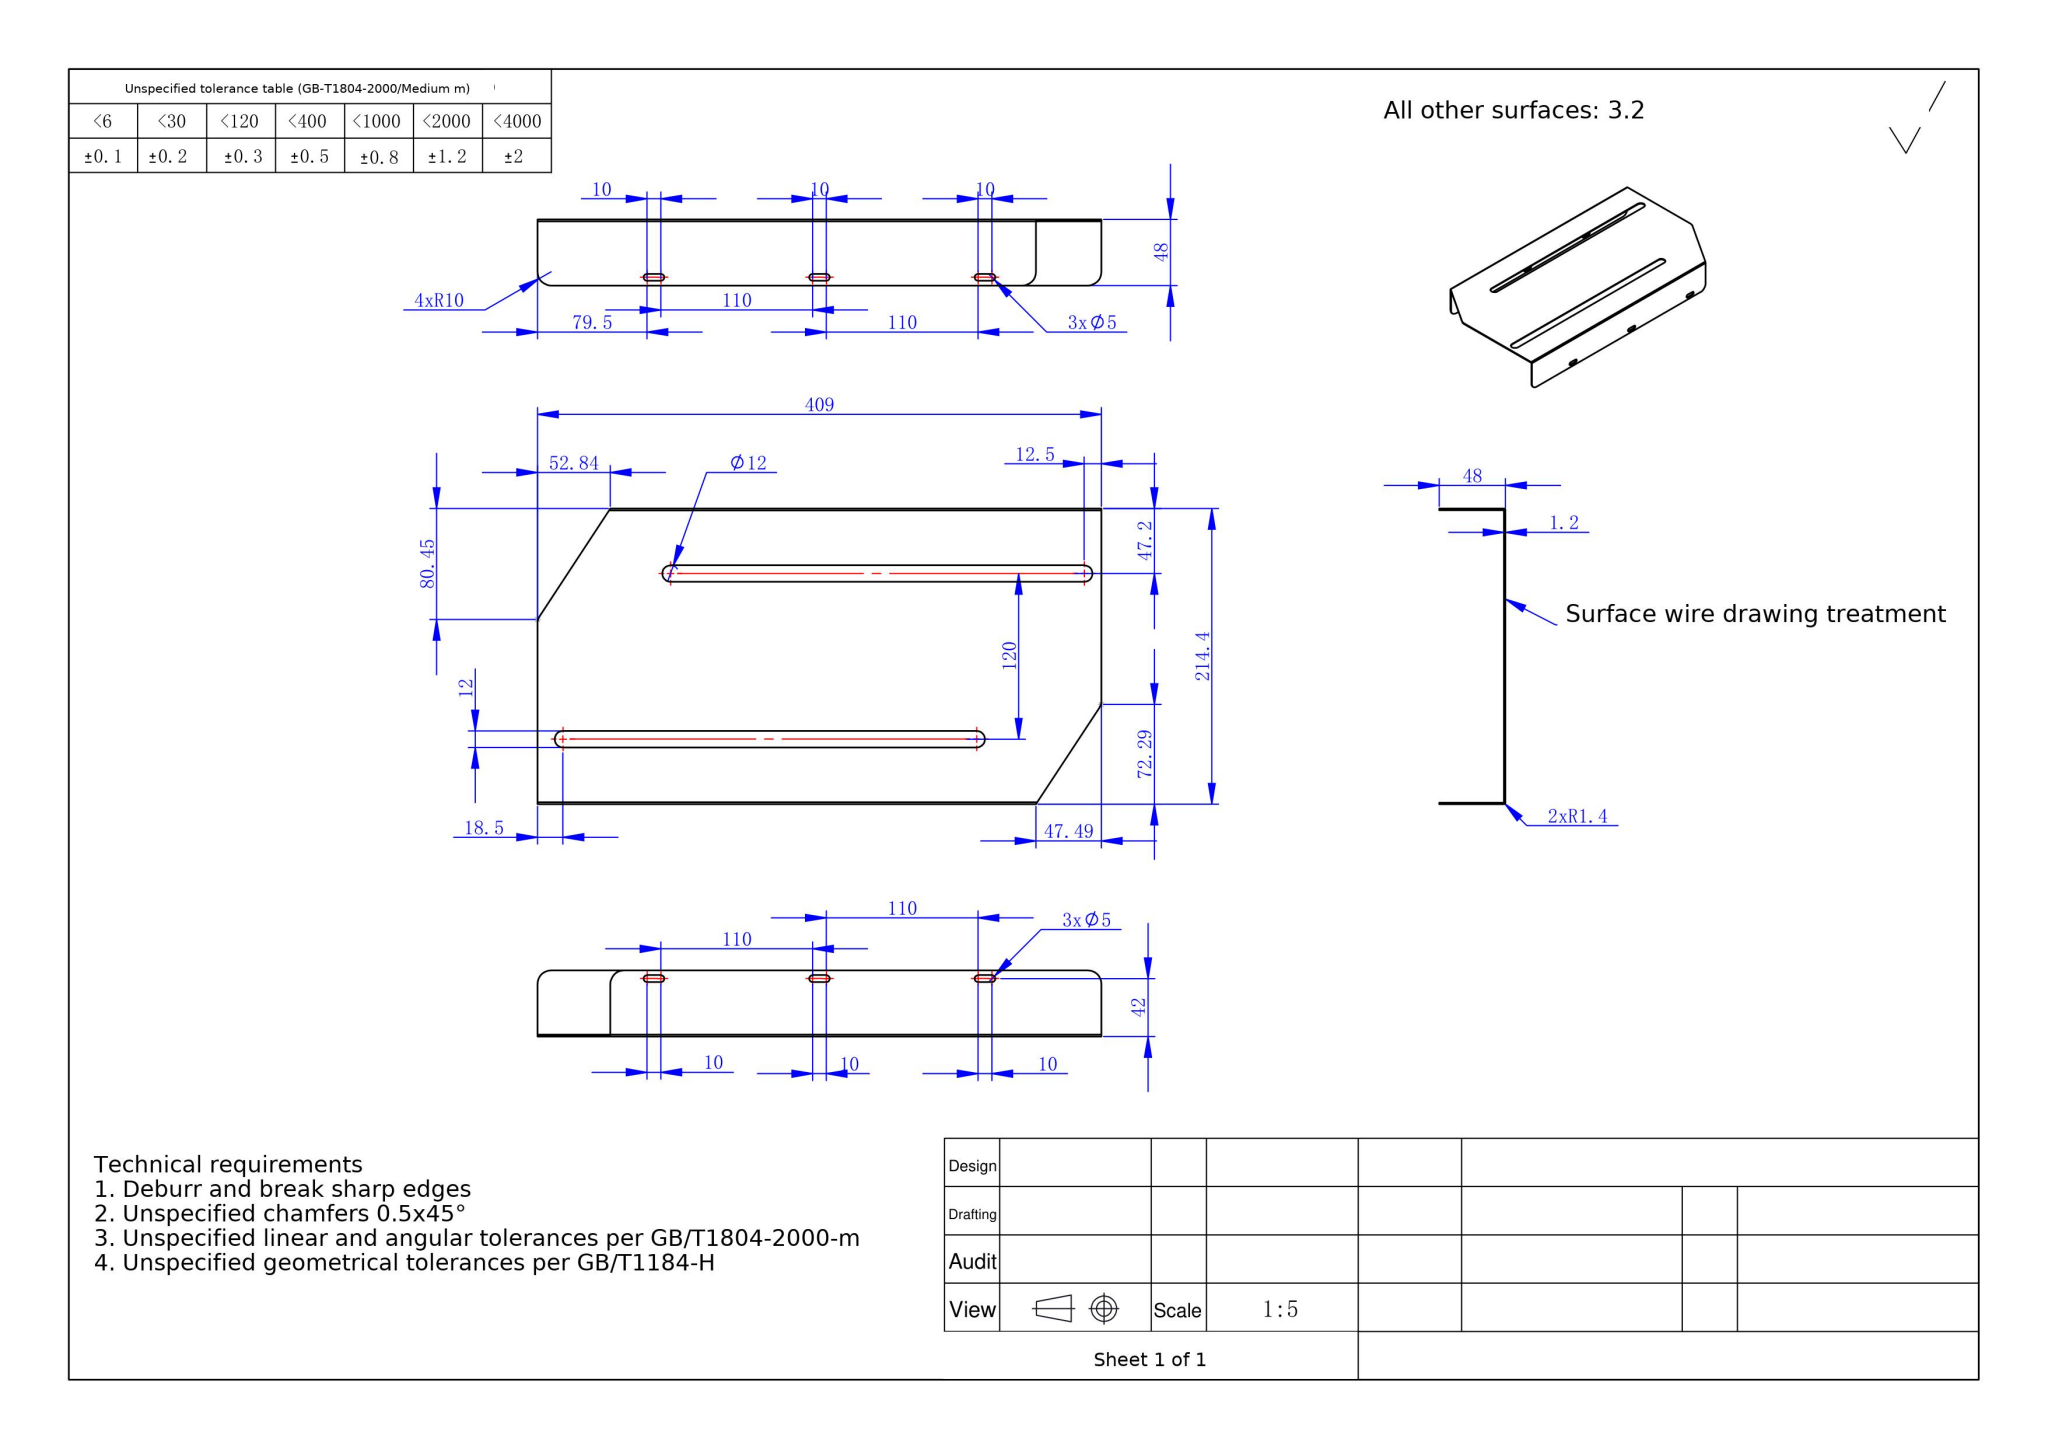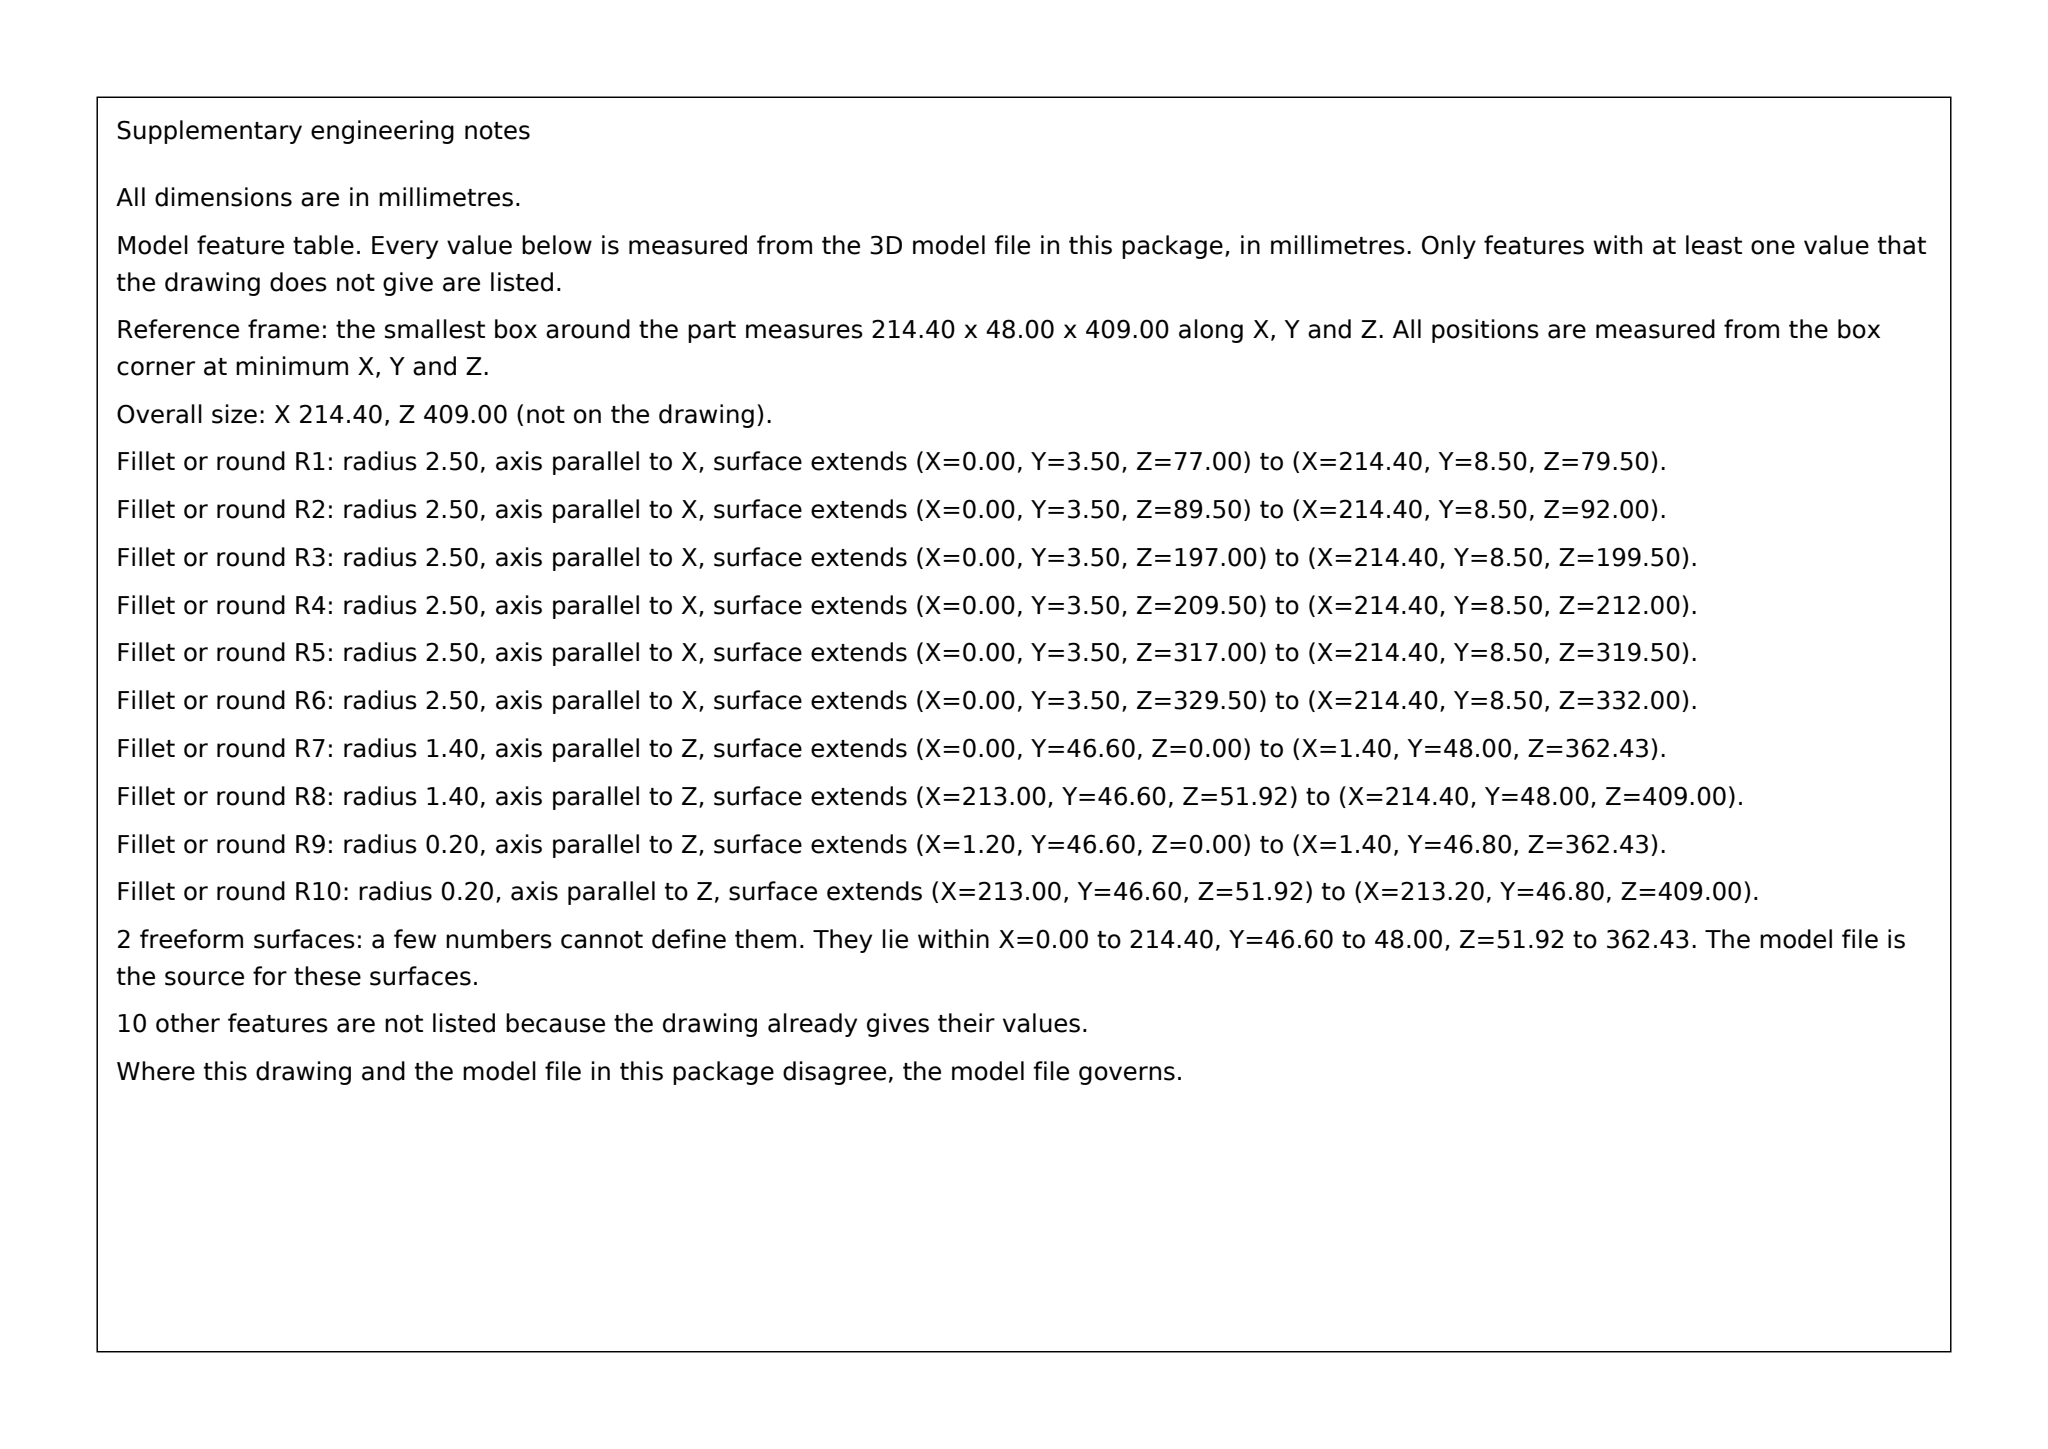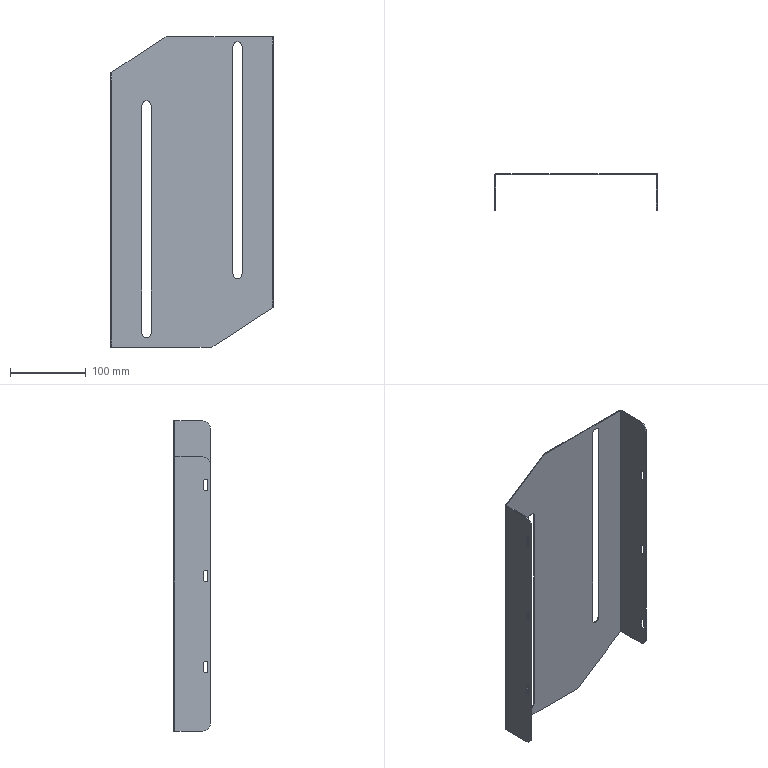Part | SolidWorks | mm | 1 solid | 64 faces | box 214.4 x 48 x 409 mm | volume 131108 mm3 | plane 34 | cylinder 28 | spline 2 | commonest cylinder face diameters 5 x12 12 x6 20 x6 2.8 x2 0.4 x2